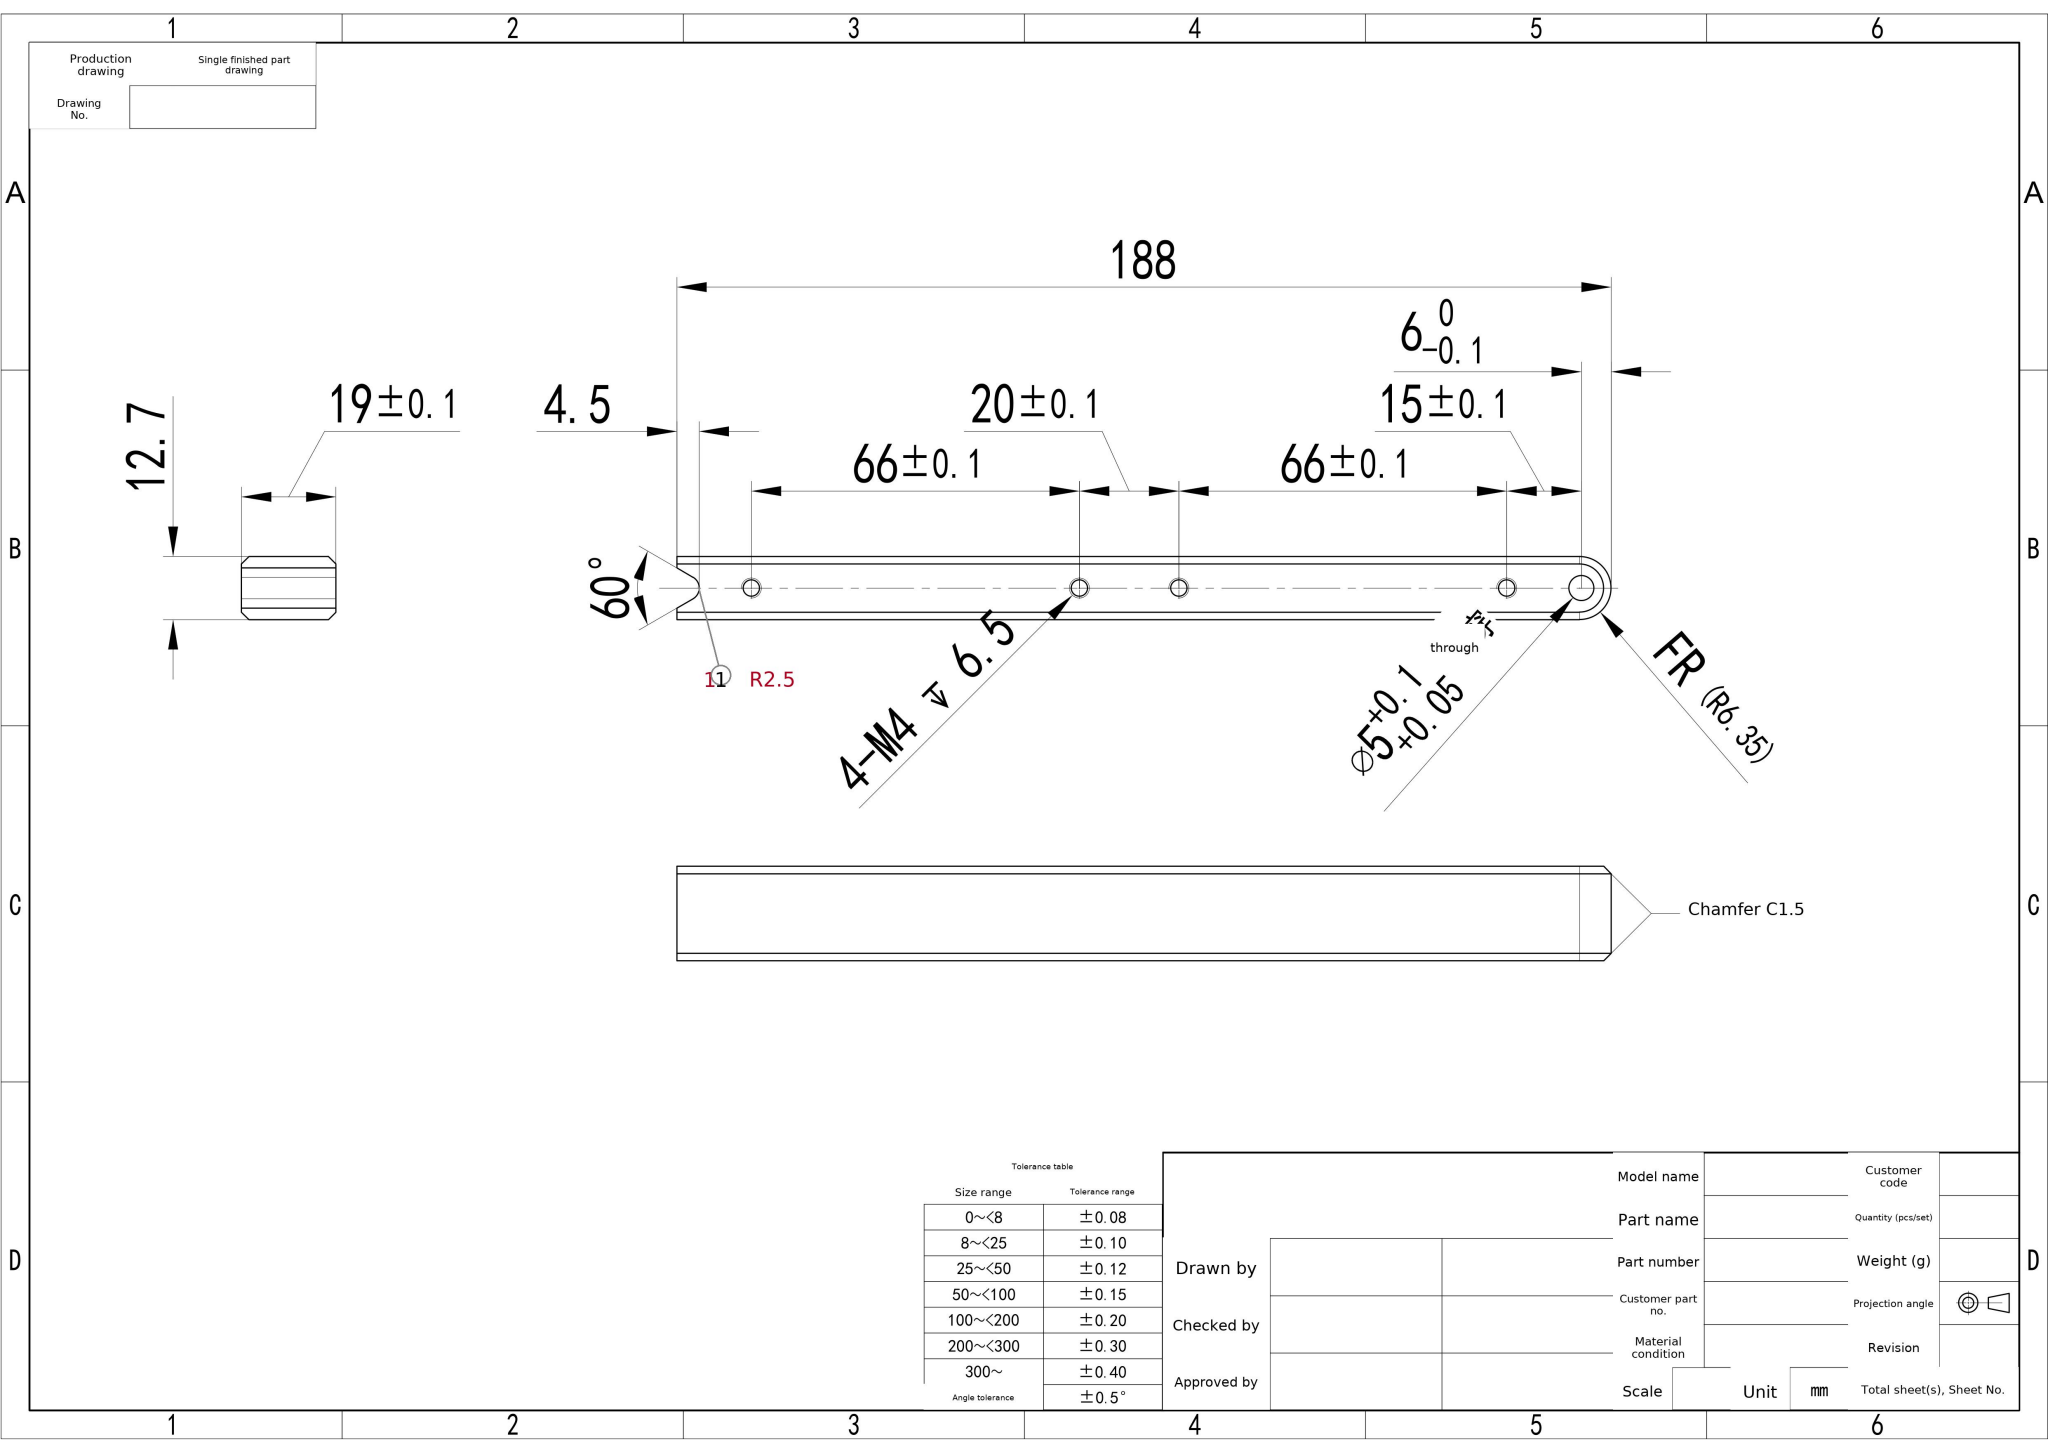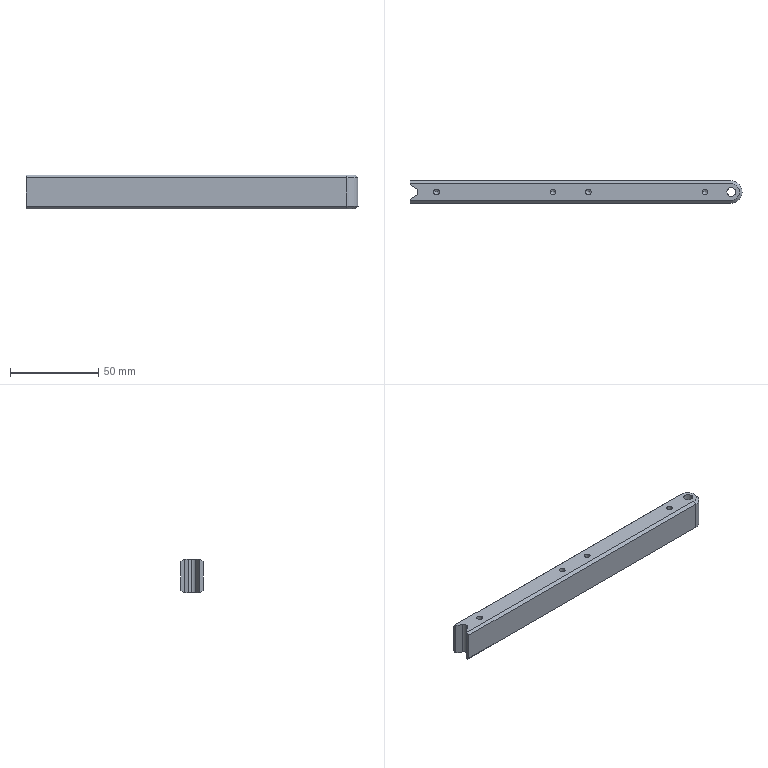Part | SolidWorks | mm | 1 solid | 37 faces | box 188 x 12.7 x 19 mm | volume 43131 mm3 | cylinder 14 | plane 12 | cone 11 | commonest cylinder face diameters 3.3 x8 5 x4 12.7 x2
STEP:
#1=CARTESIAN_POINT('',(100.65,-6.35,-17.5));
#2=VERTEX_POINT('',#1);
#3=CARTESIAN_POINT('',(107.,-0.00000002,-17.5));
#4=VERTEX_POINT('',#3);
#5=CARTESIAN_POINT('',(100.65,-0.00000002,-17.5));
#6=DIRECTION('',(0.,0.,1.));
#7=DIRECTION('',(1.,0.,0.));
#8=AXIS2_PLACEMENT_3D('',#5,#6,#7);
#9=CIRCLE('',#8,6.35);
#10=EDGE_CURVE('',#2,#4,#9,.T.);
#11=ORIENTED_EDGE('',*,*,#10,.T.);
#12=CARTESIAN_POINT('',(107.,-0.00000002,-1.5));
#13=VERTEX_POINT('',#12);
#14=CARTESIAN_POINT('',(107.,-0.00000002,-234.));
#15=DIRECTION('',(0.,0.,1.));
#16=VECTOR('',#15,1000.);
#17=LINE('',#14,#16);
#18=EDGE_CURVE('',#4,#13,#17,.T.);
#19=ORIENTED_EDGE('',*,*,#18,.T.);
#20=CARTESIAN_POINT('',(100.65,-6.35,-1.5));
#21=VERTEX_POINT('',#20);
#22=CARTESIAN_POINT('',(100.65,-0.00000002,-1.5));
#23=DIRECTION('',(0.,0.,-1.));
#24=DIRECTION('',(1.,0.,0.));
#25=AXIS2_PLACEMENT_3D('',#22,#23,#24);
#26=CIRCLE('',#25,6.35);
#27=EDGE_CURVE('',#13,#21,#26,.T.);
#28=ORIENTED_EDGE('',*,*,#27,.T.);
#29=CARTESIAN_POINT('',(100.65,-6.35,-234.));
#30=DIRECTION('',(0.,0.,-1.));
#31=VECTOR('',#30,1000.);
#32=LINE('',#29,#31);
#33=EDGE_CURVE('',#21,#2,#32,.T.);
#34=ORIENTED_EDGE('',*,*,#33,.T.);
#35=EDGE_LOOP('',(#11,#19,#28,#34));
#36=FACE_OUTER_BOUND('',#35,.T.);
#37=CARTESIAN_POINT('',(100.65,-0.00000002,-234.));
#38=DIRECTION('',(0.,0.,1.));
#39=DIRECTION('',(1.,0.,0.));
#40=AXIS2_PLACEMENT_3D('',#37,#38,#39);
#41=CYLINDRICAL_SURFACE('',#40,6.35);
#42=ADVANCED_FACE('',(#36),#41,.T.);
#43=CARTESIAN_POINT('',(105.5,-0.00000002,-19.));
#44=VERTEX_POINT('',#43);
#45=CARTESIAN_POINT('',(100.65,-4.85,-19.));
#46=VERTEX_POINT('',#45);
#47=CARTESIAN_POINT('',(100.65,-0.00000002,-19.));
#48=DIRECTION('',(0.,0.,-1.));
#49=DIRECTION('',(1.,0.,0.));
#50=AXIS2_PLACEMENT_3D('',#47,#48,#49);
#51=CIRCLE('',#50,4.85);
#52=EDGE_CURVE('',#44,#46,#51,.T.);
#53=ORIENTED_EDGE('',*,*,#52,.F.);
#54=CARTESIAN_POINT('',(107.,-0.00000002,-17.5));
#55=DIRECTION('',(0.7071,0.,0.7071));
#56=VECTOR('',#55,1000.);
#57=LINE('',#54,#56);
#58=EDGE_CURVE('',#44,#4,#57,.T.);
#59=ORIENTED_EDGE('',*,*,#58,.T.);
#60=ORIENTED_EDGE('',*,*,#10,.F.);
#61=CARTESIAN_POINT('',(100.65,-498899.35,498875.501));
#62=DIRECTION('',(0.,0.7071,-0.7071));
#63=VECTOR('',#62,1000.);
#64=LINE('',#61,#63);
#65=EDGE_CURVE('',#2,#46,#64,.T.);
#66=ORIENTED_EDGE('',*,*,#65,.T.);
#67=EDGE_LOOP('',(#53,#59,#60,#66));
#68=FACE_OUTER_BOUND('',#67,.T.);
#69=CARTESIAN_POINT('',(100.65,-0.00000002,-17.5));
#70=DIRECTION('',(0.,0.,1.));
#71=DIRECTION('',(1.,0.,0.));
#72=AXIS2_PLACEMENT_3D('',#69,#70,#71);
#73=CONICAL_SURFACE('',#72,6.35,0.7854);
#74=ADVANCED_FACE('',(#68),#73,.T.);
#75=CARTESIAN_POINT('',(-76.5,-0.,-19.));
#76=VERTEX_POINT('',#75);
#77=CARTESIAN_POINT('',(-77.75,2.165,-19.));
#78=VERTEX_POINT('',#77);
#79=CARTESIAN_POINT('',(-79.,-0.,-19.));
#80=DIRECTION('',(0.,0.,1.));
#81=DIRECTION('',(1.,0.,0.));
#82=AXIS2_PLACEMENT_3D('',#79,#80,#81);
#83=CIRCLE('',#82,2.5);
#84=EDGE_CURVE('',#76,#78,#83,.T.);
#85=ORIENTED_EDGE('',*,*,#84,.F.);
#86=CARTESIAN_POINT('',(-76.5,-0.,0.));
#87=VERTEX_POINT('',#86);
#88=CARTESIAN_POINT('',(-76.5,-0.,-234.));
#89=DIRECTION('',(0.,0.,1.));
#90=VECTOR('',#89,1000.);
#91=LINE('',#88,#90);
#92=EDGE_CURVE('',#76,#87,#91,.T.);
#93=ORIENTED_EDGE('',*,*,#92,.T.);
#94=CARTESIAN_POINT('',(-77.75,2.165,0.));
#95=VERTEX_POINT('',#94);
#96=CARTESIAN_POINT('',(-79.,-0.,0.));
#97=DIRECTION('',(0.,0.,-1.));
#98=DIRECTION('',(1.,0.,0.));
#99=AXIS2_PLACEMENT_3D('',#96,#97,#98);
#100=CIRCLE('',#99,2.5);
#101=EDGE_CURVE('',#95,#87,#100,.T.);
#102=ORIENTED_EDGE('',*,*,#101,.F.);
#103=CARTESIAN_POINT('',(-77.75,2.165,-234.));
#104=DIRECTION('',(0.,0.,-1.));
#105=VECTOR('',#104,1000.);
#106=LINE('',#103,#105);
#107=EDGE_CURVE('',#95,#78,#106,.T.);
#108=ORIENTED_EDGE('',*,*,#107,.T.);
#109=EDGE_LOOP('',(#85,#93,#102,#108));
#110=FACE_OUTER_BOUND('',#109,.T.);
#111=CARTESIAN_POINT('',(-79.,-0.,-234.));
#112=DIRECTION('',(0.,0.,1.));
#113=DIRECTION('',(1.,0.,0.));
#114=AXIS2_PLACEMENT_3D('',#111,#112,#113);
#115=CYLINDRICAL_SURFACE('',#114,2.5);
#116=ADVANCED_FACE('',(#110),#115,.F.);
#117=CARTESIAN_POINT('',(-64.35,-0.,0.));
#118=VERTEX_POINT('',#117);
#119=CARTESIAN_POINT('',(-67.65,-0.,0.));
#120=VERTEX_POINT('',#119);
#121=CARTESIAN_POINT('',(-66.,-0.,0.));
#122=DIRECTION('',(0.,0.,-1.));
#123=DIRECTION('',(-1.,0.,0.));
#124=AXIS2_PLACEMENT_3D('',#121,#122,#123);
#125=CIRCLE('',#124,1.65);
#126=EDGE_CURVE('',#118,#120,#125,.T.);
#127=ORIENTED_EDGE('',*,*,#126,.F.);
#128=CARTESIAN_POINT('',(-64.35,-0.,-6.));
#129=VERTEX_POINT('',#128);
#130=CARTESIAN_POINT('',(-64.35,-0.,0.));
#131=DIRECTION('',(0.,0.,-1.));
#132=VECTOR('',#131,1000.);
#133=LINE('',#130,#132);
#134=EDGE_CURVE('',#118,#129,#133,.T.);
#135=ORIENTED_EDGE('',*,*,#134,.T.);
#136=CARTESIAN_POINT('',(-67.65,-0.,-6.));
#137=VERTEX_POINT('',#136);
#138=CARTESIAN_POINT('',(-66.,-0.,-6.));
#139=DIRECTION('',(0.,0.,1.));
#140=DIRECTION('',(-1.,0.,0.));
#141=AXIS2_PLACEMENT_3D('',#138,#139,#140);
#142=CIRCLE('',#141,1.65);
#143=EDGE_CURVE('',#137,#129,#142,.T.);
#144=ORIENTED_EDGE('',*,*,#143,.F.);
#145=CARTESIAN_POINT('',(-67.65,-0.,0.));
#146=DIRECTION('',(0.,0.,-1.));
#147=VECTOR('',#146,1000.);
#148=LINE('',#145,#147);
#149=EDGE_CURVE('',#120,#137,#148,.T.);
#150=ORIENTED_EDGE('',*,*,#149,.F.);
#151=EDGE_LOOP('',(#127,#135,#144,#150));
#152=FACE_OUTER_BOUND('',#151,.T.);
#153=CARTESIAN_POINT('',(-66.,-0.,0.));
#154=DIRECTION('',(0.,0.,-1.));
#155=DIRECTION('',(-1.,0.,0.));
#156=AXIS2_PLACEMENT_3D('',#153,#154,#155);
#157=CYLINDRICAL_SURFACE('',#156,1.65);
#158=ADVANCED_FACE('',(#152),#157,.F.);
#159=CARTESIAN_POINT('',(1.65,0.,0.));
#160=VERTEX_POINT('',#159);
#161=CARTESIAN_POINT('',(-1.65,0.,0.));
#162=VERTEX_POINT('',#161);
#163=CARTESIAN_POINT('',(0.,0.,0.));
#164=DIRECTION('',(0.,0.,-1.));
#165=DIRECTION('',(-1.,0.,0.));
#166=AXIS2_PLACEMENT_3D('',#163,#164,#165);
#167=CIRCLE('',#166,1.65);
#168=EDGE_CURVE('',#160,#162,#167,.T.);
#169=ORIENTED_EDGE('',*,*,#168,.F.);
#170=CARTESIAN_POINT('',(1.65,0.,-6.));
#171=VERTEX_POINT('',#170);
#172=CARTESIAN_POINT('',(1.65,0.,0.));
#173=DIRECTION('',(0.,0.,-1.));
#174=VECTOR('',#173,1000.);
#175=LINE('',#172,#174);
#176=EDGE_CURVE('',#160,#171,#175,.T.);
#177=ORIENTED_EDGE('',*,*,#176,.T.);
#178=CARTESIAN_POINT('',(-1.65,0.,-6.));
#179=VERTEX_POINT('',#178);
#180=CARTESIAN_POINT('',(0.,0.,-6.));
#181=DIRECTION('',(0.,0.,1.));
#182=DIRECTION('',(-1.,0.,0.));
#183=AXIS2_PLACEMENT_3D('',#180,#181,#182);
#184=CIRCLE('',#183,1.65);
#185=EDGE_CURVE('',#179,#171,#184,.T.);
#186=ORIENTED_EDGE('',*,*,#185,.F.);
#187=CARTESIAN_POINT('',(-1.65,0.,0.));
#188=DIRECTION('',(0.,0.,-1.));
#189=VECTOR('',#188,1000.);
#190=LINE('',#187,#189);
#191=EDGE_CURVE('',#162,#179,#190,.T.);
#192=ORIENTED_EDGE('',*,*,#191,.F.);
#193=EDGE_LOOP('',(#169,#177,#186,#192));
#194=FACE_OUTER_BOUND('',#193,.T.);
#195=CARTESIAN_POINT('',(0.,0.,0.));
#196=DIRECTION('',(0.,0.,-1.));
#197=DIRECTION('',(-1.,0.,0.));
#198=AXIS2_PLACEMENT_3D('',#195,#196,#197);
#199=CYLINDRICAL_SURFACE('',#198,1.65);
#200=ADVANCED_FACE('',(#194),#199,.F.);
#201=CARTESIAN_POINT('',(21.65,0.,0.));
#202=VERTEX_POINT('',#201);
#203=CARTESIAN_POINT('',(18.35,0.,0.));
#204=VERTEX_POINT('',#203);
#205=CARTESIAN_POINT('',(20.,0.,0.));
#206=DIRECTION('',(0.,0.,-1.));
#207=DIRECTION('',(-1.,0.,0.));
#208=AXIS2_PLACEMENT_3D('',#205,#206,#207);
#209=CIRCLE('',#208,1.65);
#210=EDGE_CURVE('',#202,#204,#209,.T.);
#211=ORIENTED_EDGE('',*,*,#210,.F.);
#212=CARTESIAN_POINT('',(21.65,0.,-6.));
#213=VERTEX_POINT('',#212);
#214=CARTESIAN_POINT('',(21.65,0.,0.));
#215=DIRECTION('',(0.,0.,-1.));
#216=VECTOR('',#215,1000.);
#217=LINE('',#214,#216);
#218=EDGE_CURVE('',#202,#213,#217,.T.);
#219=ORIENTED_EDGE('',*,*,#218,.T.);
#220=CARTESIAN_POINT('',(18.35,0.,-6.));
#221=VERTEX_POINT('',#220);
#222=CARTESIAN_POINT('',(20.,0.,-6.));
#223=DIRECTION('',(0.,0.,1.));
#224=DIRECTION('',(-1.,0.,0.));
#225=AXIS2_PLACEMENT_3D('',#222,#223,#224);
#226=CIRCLE('',#225,1.65);
#227=EDGE_CURVE('',#221,#213,#226,.T.);
#228=ORIENTED_EDGE('',*,*,#227,.F.);
#229=CARTESIAN_POINT('',(18.35,0.,0.));
#230=DIRECTION('',(0.,0.,-1.));
#231=VECTOR('',#230,1000.);
#232=LINE('',#229,#231);
#233=EDGE_CURVE('',#204,#221,#232,.T.);
#234=ORIENTED_EDGE('',*,*,#233,.F.);
#235=EDGE_LOOP('',(#211,#219,#228,#234));
#236=FACE_OUTER_BOUND('',#235,.T.);
#237=CARTESIAN_POINT('',(20.,0.,0.));
#238=DIRECTION('',(0.,0.,-1.));
#239=DIRECTION('',(-1.,0.,0.));
#240=AXIS2_PLACEMENT_3D('',#237,#238,#239);
#241=CYLINDRICAL_SURFACE('',#240,1.65);
#242=ADVANCED_FACE('',(#236),#241,.F.);
#243=CARTESIAN_POINT('',(87.65,0.,0.));
#244=VERTEX_POINT('',#243);
#245=CARTESIAN_POINT('',(84.35,0.,0.));
#246=VERTEX_POINT('',#245);
#247=CARTESIAN_POINT('',(86.,0.,0.));
#248=DIRECTION('',(0.,0.,-1.));
#249=DIRECTION('',(-1.,0.,0.));
#250=AXIS2_PLACEMENT_3D('',#247,#248,#249);
#251=CIRCLE('',#250,1.65);
#252=EDGE_CURVE('',#244,#246,#251,.T.);
#253=ORIENTED_EDGE('',*,*,#252,.F.);
#254=CARTESIAN_POINT('',(87.65,0.,-6.));
#255=VERTEX_POINT('',#254);
#256=CARTESIAN_POINT('',(87.65,0.,0.));
#257=DIRECTION('',(0.,0.,-1.));
#258=VECTOR('',#257,1000.);
#259=LINE('',#256,#258);
#260=EDGE_CURVE('',#244,#255,#259,.T.);
#261=ORIENTED_EDGE('',*,*,#260,.T.);
#262=CARTESIAN_POINT('',(84.35,0.,-6.));
#263=VERTEX_POINT('',#262);
#264=CARTESIAN_POINT('',(86.,0.,-6.));
#265=DIRECTION('',(0.,0.,1.));
#266=DIRECTION('',(-1.,0.,0.));
#267=AXIS2_PLACEMENT_3D('',#264,#265,#266);
#268=CIRCLE('',#267,1.65);
#269=EDGE_CURVE('',#263,#255,#268,.T.);
#270=ORIENTED_EDGE('',*,*,#269,.F.);
#271=CARTESIAN_POINT('',(84.35,0.,0.));
#272=DIRECTION('',(0.,0.,-1.));
#273=VECTOR('',#272,1000.);
#274=LINE('',#271,#273);
#275=EDGE_CURVE('',#246,#263,#274,.T.);
#276=ORIENTED_EDGE('',*,*,#275,.F.);
#277=EDGE_LOOP('',(#253,#261,#270,#276));
#278=FACE_OUTER_BOUND('',#277,.T.);
#279=CARTESIAN_POINT('',(86.,0.,0.));
#280=DIRECTION('',(0.,0.,-1.));
#281=DIRECTION('',(-1.,0.,0.));
#282=AXIS2_PLACEMENT_3D('',#279,#280,#281);
#283=CYLINDRICAL_SURFACE('',#282,1.65);
#284=ADVANCED_FACE('',(#278),#283,.F.);
#285=CARTESIAN_POINT('',(103.5,0.,0.));
#286=VERTEX_POINT('',#285);
#287=CARTESIAN_POINT('',(98.5,0.,0.));
#288=VERTEX_POINT('',#287);
#289=CARTESIAN_POINT('',(101.,0.,0.));
#290=DIRECTION('',(0.,0.,-1.));
#291=DIRECTION('',(-1.,0.,0.));
#292=AXIS2_PLACEMENT_3D('',#289,#290,#291);
#293=CIRCLE('',#292,2.5);
#294=EDGE_CURVE('',#286,#288,#293,.T.);
#295=ORIENTED_EDGE('',*,*,#294,.F.);
#296=CARTESIAN_POINT('',(103.5,0.,-19.));
#297=VERTEX_POINT('',#296);
#298=CARTESIAN_POINT('',(103.5,0.,0.));
#299=DIRECTION('',(0.,0.,-1.));
#300=VECTOR('',#299,1000.);
#301=LINE('',#298,#300);
#302=EDGE_CURVE('',#286,#297,#301,.T.);
#303=ORIENTED_EDGE('',*,*,#302,.T.);
#304=CARTESIAN_POINT('',(98.5,0.,-19.));
#305=VERTEX_POINT('',#304);
#306=CARTESIAN_POINT('',(101.,0.,-19.));
#307=DIRECTION('',(0.,0.,1.));
#308=DIRECTION('',(-1.,0.,0.));
#309=AXIS2_PLACEMENT_3D('',#306,#307,#308);
#310=CIRCLE('',#309,2.5);
#311=EDGE_CURVE('',#305,#297,#310,.T.);
#312=ORIENTED_EDGE('',*,*,#311,.F.);
#313=CARTESIAN_POINT('',(98.5,0.,0.));
#314=DIRECTION('',(0.,0.,-1.));
#315=VECTOR('',#314,1000.);
#316=LINE('',#313,#315);
#317=EDGE_CURVE('',#288,#305,#316,.T.);
#318=ORIENTED_EDGE('',*,*,#317,.F.);
#319=EDGE_LOOP('',(#295,#303,#312,#318));
#320=FACE_OUTER_BOUND('',#319,.T.);
#321=CARTESIAN_POINT('',(101.,0.,0.));
#322=DIRECTION('',(0.,0.,-1.));
#323=DIRECTION('',(-1.,0.,0.));
#324=AXIS2_PLACEMENT_3D('',#321,#322,#323);
#325=CYLINDRICAL_SURFACE('',#324,2.5);
#326=ADVANCED_FACE('',(#320),#325,.F.);
#327=CARTESIAN_POINT('',(-66.,-0.,-6.991));
#328=VERTEX_POINT('',#327);
#329=CARTESIAN_POINT('',(-64.35,-0.,-6.));
#330=DIRECTION('',(0.8572,0.,0.515));
#331=VECTOR('',#330,1000.);
#332=LINE('',#329,#331);
#333=EDGE_CURVE('',#328,#129,#332,.T.);
#334=ORIENTED_EDGE('',*,*,#333,.F.);
#335=CARTESIAN_POINT('',(-67.65,-0.,-6.));
#336=DIRECTION('',(-0.8572,0.,0.515));
#337=VECTOR('',#336,1000.);
#338=LINE('',#335,#337);
#339=EDGE_CURVE('',#328,#137,#338,.T.);
#340=ORIENTED_EDGE('',*,*,#339,.T.);
#341=ORIENTED_EDGE('',*,*,#143,.T.);
#342=EDGE_LOOP('',(#334,#340,#341));
#343=FACE_OUTER_BOUND('',#342,.T.);
#344=CARTESIAN_POINT('',(-66.,-0.,-6.));
#345=DIRECTION('',(0.,0.,1.));
#346=DIRECTION('',(1.,0.,0.));
#347=AXIS2_PLACEMENT_3D('',#344,#345,#346);
#348=CONICAL_SURFACE('',#347,1.65,1.03);
#349=ADVANCED_FACE('',(#343),#348,.F.);
#350=CARTESIAN_POINT('',(-0.,0.,-6.991));
#351=VERTEX_POINT('',#350);
#352=CARTESIAN_POINT('',(1.65,0.,-6.));
#353=DIRECTION('',(0.8572,0.,0.515));
#354=VECTOR('',#353,1000.);
#355=LINE('',#352,#354);
#356=EDGE_CURVE('',#351,#171,#355,.T.);
#357=ORIENTED_EDGE('',*,*,#356,.F.);
#358=CARTESIAN_POINT('',(-1.65,0.,-6.));
#359=DIRECTION('',(-0.8572,0.,0.515));
#360=VECTOR('',#359,1000.);
#361=LINE('',#358,#360);
#362=EDGE_CURVE('',#351,#179,#361,.T.);
#363=ORIENTED_EDGE('',*,*,#362,.T.);
#364=ORIENTED_EDGE('',*,*,#185,.T.);
#365=EDGE_LOOP('',(#357,#363,#364));
#366=FACE_OUTER_BOUND('',#365,.T.);
#367=CARTESIAN_POINT('',(0.,0.,-6.));
#368=DIRECTION('',(0.,0.,1.));
#369=DIRECTION('',(1.,0.,0.));
#370=AXIS2_PLACEMENT_3D('',#367,#368,#369);
#371=CONICAL_SURFACE('',#370,1.65,1.03);
#372=ADVANCED_FACE('',(#366),#371,.F.);
#373=CARTESIAN_POINT('',(20.,0.,-6.991));
#374=VERTEX_POINT('',#373);
#375=CARTESIAN_POINT('',(21.65,0.,-6.));
#376=DIRECTION('',(0.8572,0.,0.515));
#377=VECTOR('',#376,1000.);
#378=LINE('',#375,#377);
#379=EDGE_CURVE('',#374,#213,#378,.T.);
#380=ORIENTED_EDGE('',*,*,#379,.F.);
#381=CARTESIAN_POINT('',(18.35,0.,-6.));
#382=DIRECTION('',(-0.8572,0.,0.515));
#383=VECTOR('',#382,1000.);
#384=LINE('',#381,#383);
#385=EDGE_CURVE('',#374,#221,#384,.T.);
#386=ORIENTED_EDGE('',*,*,#385,.T.);
#387=ORIENTED_EDGE('',*,*,#227,.T.);
#388=EDGE_LOOP('',(#380,#386,#387));
#389=FACE_OUTER_BOUND('',#388,.T.);
#390=CARTESIAN_POINT('',(20.,0.,-6.));
#391=DIRECTION('',(0.,0.,1.));
#392=DIRECTION('',(1.,0.,0.));
#393=AXIS2_PLACEMENT_3D('',#390,#391,#392);
#394=CONICAL_SURFACE('',#393,1.65,1.03);
#395=ADVANCED_FACE('',(#389),#394,.F.);
#396=CARTESIAN_POINT('',(86.,0.,-6.991));
#397=VERTEX_POINT('',#396);
#398=CARTESIAN_POINT('',(87.65,0.,-6.));
#399=DIRECTION('',(0.8572,0.,0.515));
#400=VECTOR('',#399,1000.);
#401=LINE('',#398,#400);
#402=EDGE_CURVE('',#397,#255,#401,.T.);
#403=ORIENTED_EDGE('',*,*,#402,.F.);
#404=CARTESIAN_POINT('',(84.35,0.,-6.));
#405=DIRECTION('',(-0.8572,0.,0.515));
#406=VECTOR('',#405,1000.);
#407=LINE('',#404,#406);
#408=EDGE_CURVE('',#397,#263,#407,.T.);
#409=ORIENTED_EDGE('',*,*,#408,.T.);
#410=ORIENTED_EDGE('',*,*,#269,.T.);
#411=EDGE_LOOP('',(#403,#409,#410));
#412=FACE_OUTER_BOUND('',#411,.T.);
#413=CARTESIAN_POINT('',(86.,0.,-6.));
#414=DIRECTION('',(0.,0.,1.));
#415=DIRECTION('',(1.,0.,0.));
#416=AXIS2_PLACEMENT_3D('',#413,#414,#415);
#417=CONICAL_SURFACE('',#416,1.65,1.03);
#418=ADVANCED_FACE('',(#412),#417,.F.);
#419=CARTESIAN_POINT('',(-81.,6.35,-17.5));
#420=VERTEX_POINT('',#419);
#421=CARTESIAN_POINT('',(-81.,6.35,-1.5));
#422=VERTEX_POINT('',#421);
#423=CARTESIAN_POINT('',(-81.,6.35,-1.5));
#424=DIRECTION('',(0.,0.,1.));
#425=VECTOR('',#424,1000.);
#426=LINE('',#423,#425);
#427=EDGE_CURVE('',#420,#422,#426,.T.);
#428=ORIENTED_EDGE('',*,*,#427,.T.);
#429=CARTESIAN_POINT('',(100.65,6.35,-1.5));
#430=VERTEX_POINT('',#429);
#431=CARTESIAN_POINT('',(153.,6.35,-1.5));
#432=DIRECTION('',(1.,0.,0.));
#433=VECTOR('',#432,1000.);
#434=LINE('',#431,#433);
#435=EDGE_CURVE('',#422,#430,#434,.T.);
#436=ORIENTED_EDGE('',*,*,#435,.T.);
#437=CARTESIAN_POINT('',(100.65,6.35,-17.5));
#438=VERTEX_POINT('',#437);
#439=CARTESIAN_POINT('',(100.65,6.35,-1.5));
#440=DIRECTION('',(0.,0.,-1.));
#441=VECTOR('',#440,1000.);
#442=LINE('',#439,#441);
#443=EDGE_CURVE('',#430,#438,#442,.T.);
#444=ORIENTED_EDGE('',*,*,#443,.T.);
#445=CARTESIAN_POINT('',(153.,6.35,-17.5));
#446=DIRECTION('',(-1.,0.,0.));
#447=VECTOR('',#446,1000.);
#448=LINE('',#445,#447);
#449=EDGE_CURVE('',#438,#420,#448,.T.);
#450=ORIENTED_EDGE('',*,*,#449,.T.);
#451=EDGE_LOOP('',(#428,#436,#444,#450));
#452=FACE_OUTER_BOUND('',#451,.T.);
#453=CARTESIAN_POINT('',(153.,6.35,-1.5));
#454=DIRECTION('',(0.,1.,0.));
#455=DIRECTION('',(0.,0.,1.));
#456=AXIS2_PLACEMENT_3D('',#453,#454,#455);
#457=PLANE('',#456);
#458=ADVANCED_FACE('',(#452),#457,.T.);
#459=ORIENTED_EDGE('',*,*,#435,.F.);
#460=CARTESIAN_POINT('',(-81.,4.85,0.));
#461=VERTEX_POINT('',#460);
#462=CARTESIAN_POINT('',(-81.,4.85,0.));
#463=DIRECTION('',(0.,-0.7071,0.7071));
#464=VECTOR('',#463,1000.);
#465=LINE('',#462,#464);
#466=EDGE_CURVE('',#422,#461,#465,.T.);
#467=ORIENTED_EDGE('',*,*,#466,.T.);
#468=CARTESIAN_POINT('',(100.65,4.85,-0.00000001));
#469=VERTEX_POINT('',#468);
#470=CARTESIAN_POINT('',(153.,4.85,0.));
#471=DIRECTION('',(1.,0.,0.));
#472=VECTOR('',#471,1000.);
#473=LINE('',#470,#472);
#474=EDGE_CURVE('',#461,#469,#473,.T.);
#475=ORIENTED_EDGE('',*,*,#474,.T.);
#476=CARTESIAN_POINT('',(100.65,4.85,0.));
#477=DIRECTION('',(0.,0.7071,-0.7071));
#478=VECTOR('',#477,1000.);
#479=LINE('',#476,#478);
#480=EDGE_CURVE('',#469,#430,#479,.T.);
#481=ORIENTED_EDGE('',*,*,#480,.T.);
#482=EDGE_LOOP('',(#459,#467,#475,#481));
#483=FACE_OUTER_BOUND('',#482,.T.);
#484=CARTESIAN_POINT('',(153.,4.85,0.));
#485=DIRECTION('',(0.,0.7071,0.7071));
#486=DIRECTION('',(0.,-0.7071,0.7071));
#487=AXIS2_PLACEMENT_3D('',#484,#485,#486);
#488=PLANE('',#487);
#489=ADVANCED_FACE('',(#483),#488,.T.);
#490=ORIENTED_EDGE('',*,*,#427,.F.);
#491=CARTESIAN_POINT('',(-81.,4.85,-19.));
#492=VERTEX_POINT('',#491);
#493=CARTESIAN_POINT('',(-81.,6.35,-17.5));
#494=DIRECTION('',(0.,-0.7071,-0.7071));
#495=VECTOR('',#494,1000.);
#496=LINE('',#493,#495);
#497=EDGE_CURVE('',#420,#492,#496,.T.);
#498=ORIENTED_EDGE('',*,*,#497,.T.);
#499=CARTESIAN_POINT('',(-81.,4.041,-19.));
#500=VERTEX_POINT('',#499);
#501=CARTESIAN_POINT('',(-81.,4.85,-19.));
#502=DIRECTION('',(0.,1.,0.));
#503=VECTOR('',#502,1000.);
#504=LINE('',#501,#503);
#505=EDGE_CURVE('',#500,#492,#504,.T.);
#506=ORIENTED_EDGE('',*,*,#505,.F.);
#507=CARTESIAN_POINT('',(-81.,4.041,0.));
#508=VERTEX_POINT('',#507);
#509=CARTESIAN_POINT('',(-81.,4.041,0.));
#510=DIRECTION('',(0.,0.,1.));
#511=VECTOR('',#510,1000.);
#512=LINE('',#509,#511);
#513=EDGE_CURVE('',#500,#508,#512,.T.);
#514=ORIENTED_EDGE('',*,*,#513,.T.);
#515=CARTESIAN_POINT('',(-81.,0.,0.));
#516=DIRECTION('',(0.,1.,0.));
#517=VECTOR('',#516,1000.);
#518=LINE('',#515,#517);
#519=EDGE_CURVE('',#508,#461,#518,.T.);
#520=ORIENTED_EDGE('',*,*,#519,.T.);
#521=ORIENTED_EDGE('',*,*,#466,.F.);
#522=EDGE_LOOP('',(#490,#498,#506,#514,#520,#521));
#523=FACE_OUTER_BOUND('',#522,.T.);
#524=CARTESIAN_POINT('',(-81.,0.,0.));
#525=DIRECTION('',(-1.,0.,0.));
#526=DIRECTION('',(0.,0.,1.));
#527=AXIS2_PLACEMENT_3D('',#524,#525,#526);
#528=PLANE('',#527);
#529=ADVANCED_FACE('',(#523),#528,.T.);
#530=CARTESIAN_POINT('',(100.65,4.85,-19.));
#531=VERTEX_POINT('',#530);
#532=CARTESIAN_POINT('',(153.,4.85,-19.));
#533=DIRECTION('',(-1.,0.,0.));
#534=VECTOR('',#533,1000.);
#535=LINE('',#532,#534);
#536=EDGE_CURVE('',#531,#492,#535,.T.);
#537=ORIENTED_EDGE('',*,*,#536,.T.);
#538=ORIENTED_EDGE('',*,*,#497,.F.);
#539=ORIENTED_EDGE('',*,*,#449,.F.);
#540=CARTESIAN_POINT('',(100.65,6.35,-17.5));
#541=DIRECTION('',(0.,-0.7071,-0.7071));
#542=VECTOR('',#541,1000.);
#543=LINE('',#540,#542);
#544=EDGE_CURVE('',#438,#531,#543,.T.);
#545=ORIENTED_EDGE('',*,*,#544,.T.);
#546=EDGE_LOOP('',(#537,#538,#539,#545));
#547=FACE_OUTER_BOUND('',#546,.T.);
#548=CARTESIAN_POINT('',(153.,6.35,-17.5));
#549=DIRECTION('',(0.,0.7071,-0.7071));
#550=DIRECTION('',(0.,0.7071,0.7071));
#551=AXIS2_PLACEMENT_3D('',#548,#549,#550);
#552=PLANE('',#551);
#553=ADVANCED_FACE('',(#547),#552,.T.);
#554=ORIENTED_EDGE('',*,*,#18,.F.);
#555=CARTESIAN_POINT('',(100.65,-0.00000002,-17.5));
#556=DIRECTION('',(0.,0.,1.));
#557=DIRECTION('',(1.,0.,0.));
#558=AXIS2_PLACEMENT_3D('',#555,#556,#557);
#559=CIRCLE('',#558,6.35);
#560=EDGE_CURVE('',#4,#438,#559,.T.);
#561=ORIENTED_EDGE('',*,*,#560,.T.);
#562=ORIENTED_EDGE('',*,*,#443,.F.);
#563=CARTESIAN_POINT('',(100.65,-0.00000002,-1.5));
#564=DIRECTION('',(0.,0.,-1.));
#565=DIRECTION('',(1.,0.,0.));
#566=AXIS2_PLACEMENT_3D('',#563,#564,#565);
#567=CIRCLE('',#566,6.35);
#568=EDGE_CURVE('',#430,#13,#567,.T.);
#569=ORIENTED_EDGE('',*,*,#568,.T.);
#570=EDGE_LOOP('',(#554,#561,#562,#569));
#571=FACE_OUTER_BOUND('',#570,.T.);
#572=CARTESIAN_POINT('',(100.65,-0.00000002,-234.));
#573=DIRECTION('',(0.,0.,1.));
#574=DIRECTION('',(1.,0.,0.));
#575=AXIS2_PLACEMENT_3D('',#572,#573,#574);
#576=CYLINDRICAL_SURFACE('',#575,6.35);
#577=ADVANCED_FACE('',(#571),#576,.T.);
#578=CARTESIAN_POINT('',(100.65,-4.85,-0.00000001));
#579=VERTEX_POINT('',#578);
#580=CARTESIAN_POINT('',(100.65,-499004.849,-499000.));
#581=DIRECTION('',(0.,-0.7071,-0.7071));
#582=VECTOR('',#581,1000.);
#583=LINE('',#580,#582);
#584=EDGE_CURVE('',#579,#21,#583,.T.);
#585=ORIENTED_EDGE('',*,*,#584,.T.);
#586=ORIENTED_EDGE('',*,*,#27,.F.);
#587=ORIENTED_EDGE('',*,*,#568,.F.);
#588=ORIENTED_EDGE('',*,*,#480,.F.);
#589=CARTESIAN_POINT('',(100.65,-0.00000002,-0.00000001));
#590=DIRECTION('',(0.,0.,-1.));
#591=DIRECTION('',(-1.,0.,0.));
#592=AXIS2_PLACEMENT_3D('',#589,#590,#591);
#593=CIRCLE('',#592,4.85);
#594=EDGE_CURVE('',#469,#579,#593,.T.);
#595=ORIENTED_EDGE('',*,*,#594,.T.);
#596=EDGE_LOOP('',(#585,#586,#587,#588,#595));
#597=FACE_OUTER_BOUND('',#596,.T.);
#598=CARTESIAN_POINT('',(100.65,-0.00000002,-1.5));
#599=DIRECTION('',(0.,0.,-1.));
#600=DIRECTION('',(-1.,0.,0.));
#601=AXIS2_PLACEMENT_3D('',#598,#599,#600);
#602=CONICAL_SURFACE('',#601,6.35,0.7854);
#603=ADVANCED_FACE('',(#597),#602,.T.);
#604=CARTESIAN_POINT('',(-77.75,-2.165,0.));
#605=VERTEX_POINT('',#604);
#606=CARTESIAN_POINT('',(-81.,-4.041,-0.));
#607=VERTEX_POINT('',#606);
#608=CARTESIAN_POINT('',(-77.75,-2.165,0.));
#609=DIRECTION('',(-0.866,-0.5,0.));
#610=VECTOR('',#609,1000.);
#611=LINE('',#608,#610);
#612=EDGE_CURVE('',#605,#607,#611,.T.);
#613=ORIENTED_EDGE('',*,*,#612,.T.);
#614=CARTESIAN_POINT('',(-81.,-4.85,-0.));
#615=VERTEX_POINT('',#614);
#616=CARTESIAN_POINT('',(-81.,0.,-0.));
#617=DIRECTION('',(0.,1.,0.));
#618=VECTOR('',#617,1000.);
#619=LINE('',#616,#618);
#620=EDGE_CURVE('',#615,#607,#619,.T.);
#621=ORIENTED_EDGE('',*,*,#620,.F.);
#622=CARTESIAN_POINT('',(153.,-4.85,0.));
#623=DIRECTION('',(1.,0.,0.));
#624=VECTOR('',#623,1000.);
#625=LINE('',#622,#624);
#626=EDGE_CURVE('',#615,#579,#625,.T.);
#627=ORIENTED_EDGE('',*,*,#626,.T.);
#628=ORIENTED_EDGE('',*,*,#594,.F.);
#629=ORIENTED_EDGE('',*,*,#474,.F.);
#630=ORIENTED_EDGE('',*,*,#519,.F.);
#631=CARTESIAN_POINT('',(-81.,4.041,0.));
#632=DIRECTION('',(0.866,-0.5,0.));
#633=VECTOR('',#632,1000.);
#634=LINE('',#631,#633);
#635=EDGE_CURVE('',#508,#95,#634,.T.);
#636=ORIENTED_EDGE('',*,*,#635,.T.);
#637=ORIENTED_EDGE('',*,*,#101,.T.);
#638=CARTESIAN_POINT('',(-79.,-0.,0.));
#639=DIRECTION('',(0.,0.,-1.));
#640=DIRECTION('',(1.,0.,0.));
#641=AXIS2_PLACEMENT_3D('',#638,#639,#640);
#642=CIRCLE('',#641,2.5);
#643=EDGE_CURVE('',#87,#605,#642,.T.);
#644=ORIENTED_EDGE('',*,*,#643,.T.);
#645=EDGE_LOOP('',(#613,#621,#627,#628,#629,#630,#636,#637,#644));
#646=FACE_OUTER_BOUND('',#645,.T.);
#647=CARTESIAN_POINT('',(-66.,-0.,0.));
#648=DIRECTION('',(0.,0.,-1.));
#649=DIRECTION('',(-1.,0.,0.));
#650=AXIS2_PLACEMENT_3D('',#647,#648,#649);
#651=CIRCLE('',#650,1.65);
#652=EDGE_CURVE('',#120,#118,#651,.T.);
#653=ORIENTED_EDGE('',*,*,#652,.T.);
#654=ORIENTED_EDGE('',*,*,#126,.T.);
#655=EDGE_LOOP('',(#653,#654));
#656=FACE_BOUND('',#655,.T.);
#657=CARTESIAN_POINT('',(0.,0.,0.));
#658=DIRECTION('',(0.,0.,-1.));
#659=DIRECTION('',(-1.,0.,0.));
#660=AXIS2_PLACEMENT_3D('',#657,#658,#659);
#661=CIRCLE('',#660,1.65);
#662=EDGE_CURVE('',#162,#160,#661,.T.);
#663=ORIENTED_EDGE('',*,*,#662,.T.);
#664=ORIENTED_EDGE('',*,*,#168,.T.);
#665=EDGE_LOOP('',(#663,#664));
#666=FACE_BOUND('',#665,.T.);
#667=CARTESIAN_POINT('',(20.,0.,0.));
#668=DIRECTION('',(0.,0.,-1.));
#669=DIRECTION('',(-1.,0.,0.));
#670=AXIS2_PLACEMENT_3D('',#667,#668,#669);
#671=CIRCLE('',#670,1.65);
#672=EDGE_CURVE('',#204,#202,#671,.T.);
#673=ORIENTED_EDGE('',*,*,#672,.T.);
#674=ORIENTED_EDGE('',*,*,#210,.T.);
#675=EDGE_LOOP('',(#673,#674));
#676=FACE_BOUND('',#675,.T.);
#677=CARTESIAN_POINT('',(86.,0.,0.));
#678=DIRECTION('',(0.,0.,-1.));
#679=DIRECTION('',(-1.,0.,0.));
#680=AXIS2_PLACEMENT_3D('',#677,#678,#679);
#681=CIRCLE('',#680,1.65);
#682=EDGE_CURVE('',#246,#244,#681,.T.);
#683=ORIENTED_EDGE('',*,*,#682,.T.);
#684=ORIENTED_EDGE('',*,*,#252,.T.);
#685=EDGE_LOOP('',(#683,#684));
#686=FACE_BOUND('',#685,.T.);
#687=CARTESIAN_POINT('',(101.,0.,0.));
#688=DIRECTION('',(0.,0.,-1.));
#689=DIRECTION('',(-1.,0.,0.));
#690=AXIS2_PLACEMENT_3D('',#687,#688,#689);
#691=CIRCLE('',#690,2.5);
#692=EDGE_CURVE('',#288,#286,#691,.T.);
#693=ORIENTED_EDGE('',*,*,#692,.T.);
#694=ORIENTED_EDGE('',*,*,#294,.T.);
#695=EDGE_LOOP('',(#693,#694));
#696=FACE_BOUND('',#695,.T.);
#697=CARTESIAN_POINT('',(153.,-4.85,0.));
#698=DIRECTION('',(0.,0.,1.));
#699=DIRECTION('',(1.,0.,0.));
#700=AXIS2_PLACEMENT_3D('',#697,#698,#699);
#701=PLANE('',#700);
#702=ADVANCED_FACE('',(#646,#656,#666,#676,#686,#696),#701,.T.);
#703=CARTESIAN_POINT('',(-77.75,2.165,-19.));
#704=DIRECTION('',(-0.866,0.5,0.));
#705=VECTOR('',#704,1000.);
#706=LINE('',#703,#705);
#707=EDGE_CURVE('',#78,#500,#706,.T.);
#708=ORIENTED_EDGE('',*,*,#707,.F.);
#709=ORIENTED_EDGE('',*,*,#107,.F.);
#710=ORIENTED_EDGE('',*,*,#635,.F.);
#711=ORIENTED_EDGE('',*,*,#513,.F.);
#712=EDGE_LOOP('',(#708,#709,#710,#711));
#713=FACE_OUTER_BOUND('',#712,.T.);
#714=CARTESIAN_POINT('',(-77.75,2.165,-234.));
#715=DIRECTION('',(0.5,0.866,0.));
#716=DIRECTION('',(-0.866,0.5,0.));
#717=AXIS2_PLACEMENT_3D('',#714,#715,#716);
#718=PLANE('',#717);
#719=ADVANCED_FACE('',(#713),#718,.F.);
#720=ORIENTED_EDGE('',*,*,#707,.T.);
#721=ORIENTED_EDGE('',*,*,#505,.T.);
#722=ORIENTED_EDGE('',*,*,#536,.F.);
#723=CARTESIAN_POINT('',(100.65,-0.00000002,-19.));
#724=DIRECTION('',(0.,0.,-1.));
#725=DIRECTION('',(1.,0.,0.));
#726=AXIS2_PLACEMENT_3D('',#723,#724,#725);
#727=CIRCLE('',#726,4.85);
#728=EDGE_CURVE('',#531,#44,#727,.T.);
#729=ORIENTED_EDGE('',*,*,#728,.T.);
#730=ORIENTED_EDGE('',*,*,#52,.T.);
#731=CARTESIAN_POINT('',(-81.,-4.85,-19.));
#732=VERTEX_POINT('',#731);
#733=CARTESIAN_POINT('',(153.,-4.85,-19.));
#734=DIRECTION('',(-1.,0.,0.));
#735=VECTOR('',#734,1000.);
#736=LINE('',#733,#735);
#737=EDGE_CURVE('',#46,#732,#736,.T.);
#738=ORIENTED_EDGE('',*,*,#737,.T.);
#739=CARTESIAN_POINT('',(-81.,-4.041,-19.));
#740=VERTEX_POINT('',#739);
#741=CARTESIAN_POINT('',(-81.,0.,-19.));
#742=DIRECTION('',(0.,-1.,0.));
#743=VECTOR('',#742,1000.);
#744=LINE('',#741,#743);
#745=EDGE_CURVE('',#740,#732,#744,.T.);
#746=ORIENTED_EDGE('',*,*,#745,.F.);
#747=CARTESIAN_POINT('',(-77.75,-2.165,-19.));
#748=VERTEX_POINT('',#747);
#749=CARTESIAN_POINT('',(-81.,-4.041,-19.));
#750=DIRECTION('',(0.866,0.5,0.));
#751=VECTOR('',#750,1000.);
#752=LINE('',#749,#751);
#753=EDGE_CURVE('',#740,#748,#752,.T.);
#754=ORIENTED_EDGE('',*,*,#753,.T.);
#755=CARTESIAN_POINT('',(-79.,-0.,-19.));
#756=DIRECTION('',(0.,0.,1.));
#757=DIRECTION('',(1.,0.,0.));
#758=AXIS2_PLACEMENT_3D('',#755,#756,#757);
#759=CIRCLE('',#758,2.5);
#760=EDGE_CURVE('',#748,#76,#759,.T.);
#761=ORIENTED_EDGE('',*,*,#760,.T.);
#762=ORIENTED_EDGE('',*,*,#84,.T.);
#763=EDGE_LOOP('',(#720,#721,#722,#729,#730,#738,#746,#754,#761,#762));
#764=FACE_OUTER_BOUND('',#763,.T.);
#765=ORIENTED_EDGE('',*,*,#311,.T.);
#766=CARTESIAN_POINT('',(101.,0.,-19.));
#767=DIRECTION('',(0.,0.,1.));
#768=DIRECTION('',(-1.,0.,0.));
#769=AXIS2_PLACEMENT_3D('',#766,#767,#768);
#770=CIRCLE('',#769,2.5);
#771=EDGE_CURVE('',#297,#305,#770,.T.);
#772=ORIENTED_EDGE('',*,*,#771,.T.);
#773=EDGE_LOOP('',(#765,#772));
#774=FACE_BOUND('',#773,.T.);
#775=CARTESIAN_POINT('',(153.,4.85,-19.));
#776=DIRECTION('',(0.,0.,-1.));
#777=DIRECTION('',(-1.,0.,0.));
#778=AXIS2_PLACEMENT_3D('',#775,#776,#777);
#779=PLANE('',#778);
#780=ADVANCED_FACE('',(#764,#774),#779,.T.);
#781=ORIENTED_EDGE('',*,*,#58,.F.);
#782=ORIENTED_EDGE('',*,*,#728,.F.);
#783=ORIENTED_EDGE('',*,*,#544,.F.);
#784=ORIENTED_EDGE('',*,*,#560,.F.);
#785=EDGE_LOOP('',(#781,#782,#783,#784));
#786=FACE_OUTER_BOUND('',#785,.T.);
#787=CARTESIAN_POINT('',(100.65,-0.00000002,-17.5));
#788=DIRECTION('',(0.,0.,1.));
#789=DIRECTION('',(1.,0.,0.));
#790=AXIS2_PLACEMENT_3D('',#787,#788,#789);
#791=CONICAL_SURFACE('',#790,6.35,0.7854);
#792=ADVANCED_FACE('',(#786),#791,.T.);
#793=CARTESIAN_POINT('',(-81.,-6.35,-1.5));
#794=VERTEX_POINT('',#793);
#795=CARTESIAN_POINT('',(153.,-6.35,-1.5));
#796=DIRECTION('',(-1.,0.,0.));
#797=VECTOR('',#796,1000.);
#798=LINE('',#795,#797);
#799=EDGE_CURVE('',#21,#794,#798,.T.);
#800=ORIENTED_EDGE('',*,*,#799,.T.);
#801=CARTESIAN_POINT('',(-81.,-6.35,-17.5));
#802=VERTEX_POINT('',#801);
#803=CARTESIAN_POINT('',(-81.,-6.35,-17.5));
#804=DIRECTION('',(0.,0.,-1.));
#805=VECTOR('',#804,1000.);
#806=LINE('',#803,#805);
#807=EDGE_CURVE('',#794,#802,#806,.T.);
#808=ORIENTED_EDGE('',*,*,#807,.T.);
#809=CARTESIAN_POINT('',(153.,-6.35,-17.5));
#810=DIRECTION('',(1.,0.,0.));
#811=VECTOR('',#810,1000.);
#812=LINE('',#809,#811);
#813=EDGE_CURVE('',#802,#2,#812,.T.);
#814=ORIENTED_EDGE('',*,*,#813,.T.);
#815=ORIENTED_EDGE('',*,*,#33,.F.);
#816=EDGE_LOOP('',(#800,#808,#814,#815));
#817=FACE_OUTER_BOUND('',#816,.T.);
#818=CARTESIAN_POINT('',(153.,-6.35,-17.5));
#819=DIRECTION('',(0.,-1.,0.));
#820=DIRECTION('',(0.,0.,-1.));
#821=AXIS2_PLACEMENT_3D('',#818,#819,#820);
#822=PLANE('',#821);
#823=ADVANCED_FACE('',(#817),#822,.T.);
#824=ORIENTED_EDGE('',*,*,#626,.F.);
#825=CARTESIAN_POINT('',(-81.,-6.35,-1.5));
#826=DIRECTION('',(0.,-0.7071,-0.7071));
#827=VECTOR('',#826,1000.);
#828=LINE('',#825,#827);
#829=EDGE_CURVE('',#615,#794,#828,.T.);
#830=ORIENTED_EDGE('',*,*,#829,.T.);
#831=ORIENTED_EDGE('',*,*,#799,.F.);
#832=ORIENTED_EDGE('',*,*,#584,.F.);
#833=EDGE_LOOP('',(#824,#830,#831,#832));
#834=FACE_OUTER_BOUND('',#833,.T.);
#835=CARTESIAN_POINT('',(153.,-6.35,-1.5));
#836=DIRECTION('',(0.,-0.7071,0.7071));
#837=DIRECTION('',(0.,-0.7071,-0.7071));
#838=AXIS2_PLACEMENT_3D('',#835,#836,#837);
#839=PLANE('',#838);
#840=ADVANCED_FACE('',(#834),#839,.T.);
#841=ORIENTED_EDGE('',*,*,#753,.F.);
#842=CARTESIAN_POINT('',(-81.,-4.041,-234.));
#843=DIRECTION('',(0.,0.,-1.));
#844=VECTOR('',#843,1000.);
#845=LINE('',#842,#844);
#846=EDGE_CURVE('',#607,#740,#845,.T.);
#847=ORIENTED_EDGE('',*,*,#846,.F.);
#848=ORIENTED_EDGE('',*,*,#612,.F.);
#849=CARTESIAN_POINT('',(-77.75,-2.165,-234.));
#850=DIRECTION('',(0.,0.,1.));
#851=VECTOR('',#850,1000.);
#852=LINE('',#849,#851);
#853=EDGE_CURVE('',#748,#605,#852,.T.);
#854=ORIENTED_EDGE('',*,*,#853,.F.);
#855=EDGE_LOOP('',(#841,#847,#848,#854));
#856=FACE_OUTER_BOUND('',#855,.T.);
#857=CARTESIAN_POINT('',(-81.,-4.041,-234.));
#858=DIRECTION('',(0.5,-0.866,0.));
#859=DIRECTION('',(0.866,0.5,0.));
#860=AXIS2_PLACEMENT_3D('',#857,#858,#859);
#861=PLANE('',#860);
#862=ADVANCED_FACE('',(#856),#861,.F.);
#863=ORIENTED_EDGE('',*,*,#92,.F.);
#864=ORIENTED_EDGE('',*,*,#760,.F.);
#865=ORIENTED_EDGE('',*,*,#853,.T.);
#866=ORIENTED_EDGE('',*,*,#643,.F.);
#867=EDGE_LOOP('',(#863,#864,#865,#866));
#868=FACE_OUTER_BOUND('',#867,.T.);
#869=CARTESIAN_POINT('',(-79.,-0.,-234.));
#870=DIRECTION('',(0.,0.,1.));
#871=DIRECTION('',(1.,0.,0.));
#872=AXIS2_PLACEMENT_3D('',#869,#870,#871);
#873=CYLINDRICAL_SURFACE('',#872,2.5);
#874=ADVANCED_FACE('',(#868),#873,.F.);
#875=ORIENTED_EDGE('',*,*,#134,.F.);
#876=ORIENTED_EDGE('',*,*,#652,.F.);
#877=ORIENTED_EDGE('',*,*,#149,.T.);
#878=CARTESIAN_POINT('',(-66.,-0.,-6.));
#879=DIRECTION('',(0.,0.,1.));
#880=DIRECTION('',(-1.,0.,0.));
#881=AXIS2_PLACEMENT_3D('',#878,#879,#880);
#882=CIRCLE('',#881,1.65);
#883=EDGE_CURVE('',#129,#137,#882,.T.);
#884=ORIENTED_EDGE('',*,*,#883,.F.);
#885=EDGE_LOOP('',(#875,#876,#877,#884));
#886=FACE_OUTER_BOUND('',#885,.T.);
#887=CARTESIAN_POINT('',(-66.,-0.,0.));
#888=DIRECTION('',(0.,0.,-1.));
#889=DIRECTION('',(-1.,0.,0.));
#890=AXIS2_PLACEMENT_3D('',#887,#888,#889);
#891=CYLINDRICAL_SURFACE('',#890,1.65);
#892=ADVANCED_FACE('',(#886),#891,.F.);
#893=ORIENTED_EDGE('',*,*,#176,.F.);
#894=ORIENTED_EDGE('',*,*,#662,.F.);
#895=ORIENTED_EDGE('',*,*,#191,.T.);
#896=CARTESIAN_POINT('',(0.,0.,-6.));
#897=DIRECTION('',(0.,0.,1.));
#898=DIRECTION('',(-1.,0.,0.));
#899=AXIS2_PLACEMENT_3D('',#896,#897,#898);
#900=CIRCLE('',#899,1.65);
#901=EDGE_CURVE('',#171,#179,#900,.T.);
#902=ORIENTED_EDGE('',*,*,#901,.F.);
#903=EDGE_LOOP('',(#893,#894,#895,#902));
#904=FACE_OUTER_BOUND('',#903,.T.);
#905=CARTESIAN_POINT('',(0.,0.,0.));
#906=DIRECTION('',(0.,0.,-1.));
#907=DIRECTION('',(-1.,0.,0.));
#908=AXIS2_PLACEMENT_3D('',#905,#906,#907);
#909=CYLINDRICAL_SURFACE('',#908,1.65);
#910=ADVANCED_FACE('',(#904),#909,.F.);
#911=ORIENTED_EDGE('',*,*,#218,.F.);
#912=ORIENTED_EDGE('',*,*,#672,.F.);
#913=ORIENTED_EDGE('',*,*,#233,.T.);
#914=CARTESIAN_POINT('',(20.,0.,-6.));
#915=DIRECTION('',(0.,0.,1.));
#916=DIRECTION('',(-1.,0.,0.));
#917=AXIS2_PLACEMENT_3D('',#914,#915,#916);
#918=CIRCLE('',#917,1.65);
#919=EDGE_CURVE('',#213,#221,#918,.T.);
#920=ORIENTED_EDGE('',*,*,#919,.F.);
#921=EDGE_LOOP('',(#911,#912,#913,#920));
#922=FACE_OUTER_BOUND('',#921,.T.);
#923=CARTESIAN_POINT('',(20.,0.,0.));
#924=DIRECTION('',(0.,0.,-1.));
#925=DIRECTION('',(-1.,0.,0.));
#926=AXIS2_PLACEMENT_3D('',#923,#924,#925);
#927=CYLINDRICAL_SURFACE('',#926,1.65);
#928=ADVANCED_FACE('',(#922),#927,.F.);
#929=ORIENTED_EDGE('',*,*,#260,.F.);
#930=ORIENTED_EDGE('',*,*,#682,.F.);
#931=ORIENTED_EDGE('',*,*,#275,.T.);
#932=CARTESIAN_POINT('',(86.,0.,-6.));
#933=DIRECTION('',(0.,0.,1.));
#934=DIRECTION('',(-1.,0.,0.));
#935=AXIS2_PLACEMENT_3D('',#932,#933,#934);
#936=CIRCLE('',#935,1.65);
#937=EDGE_CURVE('',#255,#263,#936,.T.);
#938=ORIENTED_EDGE('',*,*,#937,.F.);
#939=EDGE_LOOP('',(#929,#930,#931,#938));
#940=FACE_OUTER_BOUND('',#939,.T.);
#941=CARTESIAN_POINT('',(86.,0.,0.));
#942=DIRECTION('',(0.,0.,-1.));
#943=DIRECTION('',(-1.,0.,0.));
#944=AXIS2_PLACEMENT_3D('',#941,#942,#943);
#945=CYLINDRICAL_SURFACE('',#944,1.65);
#946=ADVANCED_FACE('',(#940),#945,.F.);
#947=ORIENTED_EDGE('',*,*,#302,.F.);
#948=ORIENTED_EDGE('',*,*,#692,.F.);
#949=ORIENTED_EDGE('',*,*,#317,.T.);
#950=ORIENTED_EDGE('',*,*,#771,.F.);
#951=EDGE_LOOP('',(#947,#948,#949,#950));
#952=FACE_OUTER_BOUND('',#951,.T.);
#953=CARTESIAN_POINT('',(101.,0.,0.));
#954=DIRECTION('',(0.,0.,-1.));
#955=DIRECTION('',(-1.,0.,0.));
#956=AXIS2_PLACEMENT_3D('',#953,#954,#955);
#957=CYLINDRICAL_SURFACE('',#956,2.5);
#958=ADVANCED_FACE('',(#952),#957,.F.);
#959=ORIENTED_EDGE('',*,*,#813,.F.);
#960=CARTESIAN_POINT('',(-81.,-4.85,-19.));
#961=DIRECTION('',(0.,0.7071,-0.7071));
#962=VECTOR('',#961,1000.);
#963=LINE('',#960,#962);
#964=EDGE_CURVE('',#802,#732,#963,.T.);
#965=ORIENTED_EDGE('',*,*,#964,.T.);
#966=ORIENTED_EDGE('',*,*,#737,.F.);
#967=ORIENTED_EDGE('',*,*,#65,.F.);
#968=EDGE_LOOP('',(#959,#965,#966,#967));
#969=FACE_OUTER_BOUND('',#968,.T.);
#970=CARTESIAN_POINT('',(153.,-4.85,-19.));
#971=DIRECTION('',(0.,-0.7071,-0.7071));
#972=DIRECTION('',(0.,0.7071,-0.7071));
#973=AXIS2_PLACEMENT_3D('',#970,#971,#972);
#974=PLANE('',#973);
#975=ADVANCED_FACE('',(#969),#974,.T.);
#976=ORIENTED_EDGE('',*,*,#829,.F.);
#977=ORIENTED_EDGE('',*,*,#620,.T.);
#978=ORIENTED_EDGE('',*,*,#846,.T.);
#979=ORIENTED_EDGE('',*,*,#745,.T.);
#980=ORIENTED_EDGE('',*,*,#964,.F.);
#981=ORIENTED_EDGE('',*,*,#807,.F.);
#982=EDGE_LOOP('',(#976,#977,#978,#979,#980,#981));
#983=FACE_OUTER_BOUND('',#982,.T.);
#984=CARTESIAN_POINT('',(-81.,0.,0.));
#985=DIRECTION('',(-1.,0.,0.));
#986=DIRECTION('',(0.,0.,1.));
#987=AXIS2_PLACEMENT_3D('',#984,#985,#986);
#988=PLANE('',#987);
#989=ADVANCED_FACE('',(#983),#988,.T.);
#990=ORIENTED_EDGE('',*,*,#339,.F.);
#991=ORIENTED_EDGE('',*,*,#333,.T.);
#992=ORIENTED_EDGE('',*,*,#883,.T.);
#993=EDGE_LOOP('',(#990,#991,#992));
#994=FACE_OUTER_BOUND('',#993,.T.);
#995=CARTESIAN_POINT('',(-66.,-0.,-6.));
#996=DIRECTION('',(0.,0.,1.));
#997=DIRECTION('',(1.,0.,0.));
#998=AXIS2_PLACEMENT_3D('',#995,#996,#997);
#999=CONICAL_SURFACE('',#998,1.65,1.03);
#1000=ADVANCED_FACE('',(#994),#999,.F.);
#1001=ORIENTED_EDGE('',*,*,#362,.F.);
#1002=ORIENTED_EDGE('',*,*,#356,.T.);
#1003=ORIENTED_EDGE('',*,*,#901,.T.);
#1004=EDGE_LOOP('',(#1001,#1002,#1003));
#1005=FACE_OUTER_BOUND('',#1004,.T.);
#1006=CARTESIAN_POINT('',(0.,0.,-6.));
#1007=DIRECTION('',(0.,0.,1.));
#1008=DIRECTION('',(1.,0.,0.));
#1009=AXIS2_PLACEMENT_3D('',#1006,#1007,#1008);
#1010=CONICAL_SURFACE('',#1009,1.65,1.03);
#1011=ADVANCED_FACE('',(#1005),#1010,.F.);
#1012=ORIENTED_EDGE('',*,*,#385,.F.);
#1013=ORIENTED_EDGE('',*,*,#379,.T.);
#1014=ORIENTED_EDGE('',*,*,#919,.T.);
#1015=EDGE_LOOP('',(#1012,#1013,#1014));
#1016=FACE_OUTER_BOUND('',#1015,.T.);
#1017=CARTESIAN_POINT('',(20.,0.,-6.));
#1018=DIRECTION('',(0.,0.,1.));
#1019=DIRECTION('',(1.,0.,0.));
#1020=AXIS2_PLACEMENT_3D('',#1017,#1018,#1019);
#1021=CONICAL_SURFACE('',#1020,1.65,1.03);
#1022=ADVANCED_FACE('',(#1016),#1021,.F.);
#1023=ORIENTED_EDGE('',*,*,#408,.F.);
#1024=ORIENTED_EDGE('',*,*,#402,.T.);
#1025=ORIENTED_EDGE('',*,*,#937,.T.);
#1026=EDGE_LOOP('',(#1023,#1024,#1025));
#1027=FACE_OUTER_BOUND('',#1026,.T.);
#1028=CARTESIAN_POINT('',(86.,0.,-6.));
#1029=DIRECTION('',(0.,0.,1.));
#1030=DIRECTION('',(1.,0.,0.));
#1031=AXIS2_PLACEMENT_3D('',#1028,#1029,#1030);
#1032=CONICAL_SURFACE('',#1031,1.65,1.03);
#1033=ADVANCED_FACE('',(#1027),#1032,.F.);
#1034=CLOSED_SHELL('',(#42,#74,#116,#158,#200,#242,#284,#326,#349,#372,#395,#418,#458,#489,#529,#553,#577,#603,#702,#719,#780,#792,#823,#840,#862,#874,#892,#910,#928,#946,#958,#975,#989,#1000,#1011,#1022,#1033));
#1035=MANIFOLD_SOLID_BREP('',#1034);
#1036=CARTESIAN_POINT('',(0.,0.,0.));
#1037=DIRECTION('',(0.,0.,1.));
#1038=DIRECTION('',(1.,0.,0.));
#1039=AXIS2_PLACEMENT_3D('',#1036,#1037,#1038);
#1040=(LENGTH_UNIT()NAMED_UNIT(*)SI_UNIT(.MILLI.,.METRE.));
#1041=UNCERTAINTY_MEASURE_WITH_UNIT(LENGTH_MEASURE(0.00001),#1040,'','');
#1042=(NAMED_UNIT(*)PLANE_ANGLE_UNIT()SI_UNIT($,.RADIAN.));
#1043=(NAMED_UNIT(*)SI_UNIT($,.STERADIAN.)SOLID_ANGLE_UNIT());
#1044=(GEOMETRIC_REPRESENTATION_CONTEXT(3)GLOBAL_UNCERTAINTY_ASSIGNED_CONTEXT((#1041))GLOBAL_UNIT_ASSIGNED_CONTEXT((#1040,#1042,#1043))REPRESENTATION_CONTEXT('',''));
#1045=ADVANCED_BREP_SHAPE_REPRESENTATION('',(#1035,#1039),#1044);